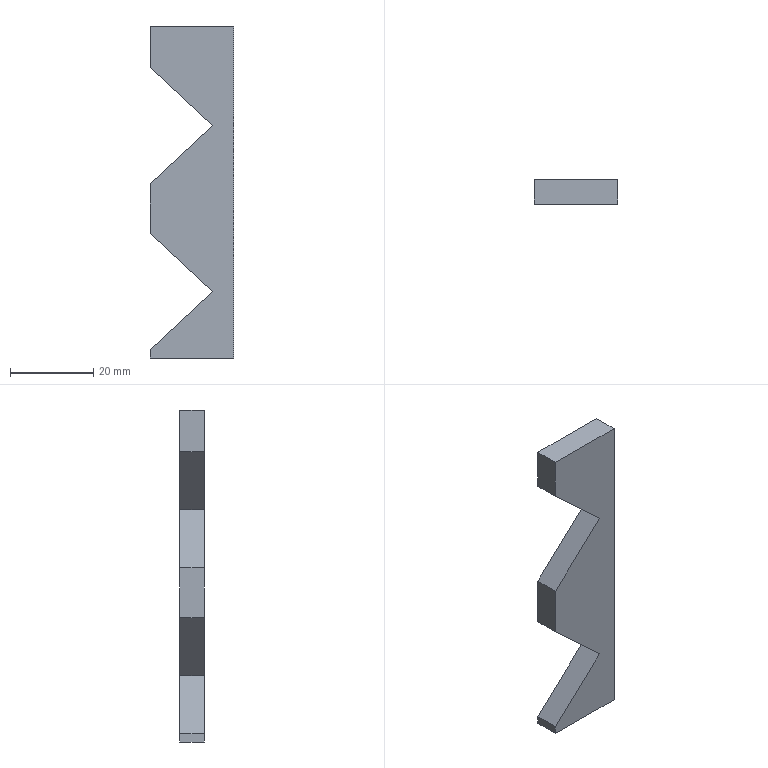Component | NX | V_SLIDER | 1 solid | 12 faces | box 20 x 6 x 80 mm | volume 7082 mm3 | plane 12
STEP:
#1=CARTESIAN_POINT('',(0.,0.,0.));
#2=DIRECTION('',(0.,0.,1.));
#3=DIRECTION('',(1.,0.,0.));
#4=AXIS2_PLACEMENT_3D('',#1,#2,#3);
#5=CARTESIAN_POINT('',(65.,-18.,99.));
#6=VERTEX_POINT('',#5);
#7=CARTESIAN_POINT('',(65.,-18.,19.));
#8=VERTEX_POINT('',#7);
#9=CARTESIAN_POINT('',(65.,-18.,99.));
#10=DIRECTION('',(0.,0.,-1.));
#11=VECTOR('',#10,1.);
#12=LINE('',#9,#11);
#13=CARTESIAN_POINT('',(65.,-12.,99.));
#14=DIRECTION('',(-1.,0.,0.));
#15=DIRECTION('',(0.,-1.,0.));
#16=AXIS2_PLACEMENT_3D('',#13,#14,#15);
#17=PLANE('',#16);
#18=CARTESIAN_POINT('',(6.,0.));
#19=DIRECTION('',(0.,-1.));
#20=VECTOR('',#19,1.);
#21=LINE('',#18,#20);
#22=(GEOMETRIC_REPRESENTATION_CONTEXT(2)PARAMETRIC_REPRESENTATION_CONTEXT()REPRESENTATION_CONTEXT('',''));
#23=DEFINITIONAL_REPRESENTATION('',(#21),#22);
#24=PCURVE('',#17,#23);
#25=CARTESIAN_POINT('',(65.,-18.,19.));
#26=DIRECTION('',(0.,1.,0.));
#27=DIRECTION('',(-1.,0.,0.));
#28=AXIS2_PLACEMENT_3D('',#25,#26,#27);
#29=PLANE('',#28);
#30=CARTESIAN_POINT('',(0.,80.));
#31=DIRECTION('',(0.,-1.));
#32=VECTOR('',#31,1.);
#33=LINE('',#30,#32);
#34=(GEOMETRIC_REPRESENTATION_CONTEXT(2)PARAMETRIC_REPRESENTATION_CONTEXT()REPRESENTATION_CONTEXT('',''));
#35=DEFINITIONAL_REPRESENTATION('',(#33),#34);
#36=PCURVE('',#29,#35);
#37=SURFACE_CURVE('',#12,(#24,#36),.PCURVE_S1.);
#38=EDGE_CURVE('',#6,#8,#37,.T.);
#39=ORIENTED_EDGE('',*,*,#38,.T.);
#40=CARTESIAN_POINT('',(65.,-12.,19.));
#41=VERTEX_POINT('',#40);
#42=CARTESIAN_POINT('',(65.,-12.,19.));
#43=DIRECTION('',(0.,-1.,0.));
#44=VECTOR('',#43,1.);
#45=LINE('',#42,#44);
#46=CARTESIAN_POINT('',(0.,-80.));
#47=DIRECTION('',(1.,0.));
#48=VECTOR('',#47,1.);
#49=LINE('',#46,#48);
#50=(GEOMETRIC_REPRESENTATION_CONTEXT(2)PARAMETRIC_REPRESENTATION_CONTEXT()REPRESENTATION_CONTEXT('',''));
#51=DEFINITIONAL_REPRESENTATION('',(#49),#50);
#52=PCURVE('',#17,#51);
#53=CARTESIAN_POINT('',(65.,-12.,19.));
#54=DIRECTION('',(-0.,0.,1.));
#55=DIRECTION('',(1.,0.,0.));
#56=AXIS2_PLACEMENT_3D('',#53,#54,#55);
#57=PLANE('',#56);
#58=CARTESIAN_POINT('',(0.,0.));
#59=DIRECTION('',(0.,-1.));
#60=VECTOR('',#59,1.);
#61=LINE('',#58,#60);
#62=(GEOMETRIC_REPRESENTATION_CONTEXT(2)PARAMETRIC_REPRESENTATION_CONTEXT()REPRESENTATION_CONTEXT('',''));
#63=DEFINITIONAL_REPRESENTATION('',(#61),#62);
#64=PCURVE('',#57,#63);
#65=SURFACE_CURVE('',#45,(#52,#64),.PCURVE_S1.);
#66=EDGE_CURVE('',#41,#8,#65,.T.);
#67=ORIENTED_EDGE('',*,*,#66,.F.);
#68=CARTESIAN_POINT('',(65.,-12.,99.));
#69=VERTEX_POINT('',#68);
#70=CARTESIAN_POINT('',(65.,-12.,99.));
#71=DIRECTION('',(0.,0.,-1.));
#72=VECTOR('',#71,1.);
#73=LINE('',#70,#72);
#74=CARTESIAN_POINT('',(0.,0.));
#75=DIRECTION('',(0.,-1.));
#76=VECTOR('',#75,1.);
#77=LINE('',#74,#76);
#78=(GEOMETRIC_REPRESENTATION_CONTEXT(2)PARAMETRIC_REPRESENTATION_CONTEXT()REPRESENTATION_CONTEXT('',''));
#79=DEFINITIONAL_REPRESENTATION('',(#77),#78);
#80=PCURVE('',#17,#79);
#81=CARTESIAN_POINT('',(65.,-12.,19.));
#82=DIRECTION('',(0.,1.,0.));
#83=DIRECTION('',(-1.,0.,0.));
#84=AXIS2_PLACEMENT_3D('',#81,#82,#83);
#85=PLANE('',#84);
#86=CARTESIAN_POINT('',(0.,80.));
#87=DIRECTION('',(0.,-1.));
#88=VECTOR('',#87,1.);
#89=LINE('',#86,#88);
#90=(GEOMETRIC_REPRESENTATION_CONTEXT(2)PARAMETRIC_REPRESENTATION_CONTEXT()REPRESENTATION_CONTEXT('',''));
#91=DEFINITIONAL_REPRESENTATION('',(#89),#90);
#92=PCURVE('',#85,#91);
#93=SURFACE_CURVE('',#73,(#80,#92),.PCURVE_S1.);
#94=EDGE_CURVE('',#69,#41,#93,.T.);
#95=ORIENTED_EDGE('',*,*,#94,.F.);
#96=CARTESIAN_POINT('',(65.,-12.,99.));
#97=DIRECTION('',(0.,-1.,0.));
#98=VECTOR('',#97,1.);
#99=LINE('',#96,#98);
#100=CARTESIAN_POINT('',(0.,0.));
#101=DIRECTION('',(1.,0.));
#102=VECTOR('',#101,1.);
#103=LINE('',#100,#102);
#104=(GEOMETRIC_REPRESENTATION_CONTEXT(2)PARAMETRIC_REPRESENTATION_CONTEXT()REPRESENTATION_CONTEXT('',''));
#105=DEFINITIONAL_REPRESENTATION('',(#103),#104);
#106=PCURVE('',#17,#105);
#107=CARTESIAN_POINT('',(45.,-12.,99.));
#108=DIRECTION('',(0.,0.,-1.));
#109=DIRECTION('',(0.,-1.,0.));
#110=AXIS2_PLACEMENT_3D('',#107,#108,#109);
#111=PLANE('',#110);
#112=CARTESIAN_POINT('',(0.,-20.));
#113=DIRECTION('',(1.,0.));
#114=VECTOR('',#113,1.);
#115=LINE('',#112,#114);
#116=(GEOMETRIC_REPRESENTATION_CONTEXT(2)PARAMETRIC_REPRESENTATION_CONTEXT()REPRESENTATION_CONTEXT('',''));
#117=DEFINITIONAL_REPRESENTATION('',(#115),#116);
#118=PCURVE('',#111,#117);
#119=SURFACE_CURVE('',#99,(#106,#118),.PCURVE_S1.);
#120=EDGE_CURVE('',#69,#6,#119,.T.);
#121=ORIENTED_EDGE('',*,*,#120,.T.);
#122=EDGE_LOOP('',(#39,#67,#95,#121));
#123=FACE_BOUND('',#122,.T.);
#124=ADVANCED_FACE('',(#123),#17,.F.);
#125=CARTESIAN_POINT('',(45.,-18.,19.));
#126=VERTEX_POINT('',#125);
#127=CARTESIAN_POINT('',(65.,-18.,19.));
#128=DIRECTION('',(-1.,0.,-0.));
#129=VECTOR('',#128,1.);
#130=LINE('',#127,#129);
#131=CARTESIAN_POINT('',(0.,-6.));
#132=DIRECTION('',(-1.,0.));
#133=VECTOR('',#132,1.);
#134=LINE('',#131,#133);
#135=(GEOMETRIC_REPRESENTATION_CONTEXT(2)PARAMETRIC_REPRESENTATION_CONTEXT()REPRESENTATION_CONTEXT('',''));
#136=DEFINITIONAL_REPRESENTATION('',(#134),#135);
#137=PCURVE('',#57,#136);
#138=CARTESIAN_POINT('',(0.,0.));
#139=DIRECTION('',(1.,-0.));
#140=VECTOR('',#139,1.);
#141=LINE('',#138,#140);
#142=(GEOMETRIC_REPRESENTATION_CONTEXT(2)PARAMETRIC_REPRESENTATION_CONTEXT()REPRESENTATION_CONTEXT('',''));
#143=DEFINITIONAL_REPRESENTATION('',(#141),#142);
#144=PCURVE('',#29,#143);
#145=SURFACE_CURVE('',#130,(#137,#144),.PCURVE_S1.);
#146=EDGE_CURVE('',#8,#126,#145,.T.);
#147=ORIENTED_EDGE('',*,*,#146,.T.);
#148=CARTESIAN_POINT('',(45.,-12.,19.));
#149=VERTEX_POINT('',#148);
#150=CARTESIAN_POINT('',(45.,-12.,19.));
#151=DIRECTION('',(0.,-1.,0.));
#152=VECTOR('',#151,1.);
#153=LINE('',#150,#152);
#154=CARTESIAN_POINT('',(-20.,0.));
#155=DIRECTION('',(0.,-1.));
#156=VECTOR('',#155,1.);
#157=LINE('',#154,#156);
#158=(GEOMETRIC_REPRESENTATION_CONTEXT(2)PARAMETRIC_REPRESENTATION_CONTEXT()REPRESENTATION_CONTEXT('',''));
#159=DEFINITIONAL_REPRESENTATION('',(#157),#158);
#160=PCURVE('',#57,#159);
#161=CARTESIAN_POINT('',(45.,-12.,19.));
#162=DIRECTION('',(1.,0.,0.));
#163=DIRECTION('',(0.,1.,0.));
#164=AXIS2_PLACEMENT_3D('',#161,#162,#163);
#165=PLANE('',#164);
#166=CARTESIAN_POINT('',(0.,0.));
#167=DIRECTION('',(-1.,0.));
#168=VECTOR('',#167,1.);
#169=LINE('',#166,#168);
#170=(GEOMETRIC_REPRESENTATION_CONTEXT(2)PARAMETRIC_REPRESENTATION_CONTEXT()REPRESENTATION_CONTEXT('',''));
#171=DEFINITIONAL_REPRESENTATION('',(#169),#170);
#172=PCURVE('',#165,#171);
#173=SURFACE_CURVE('',#153,(#160,#172),.PCURVE_S1.);
#174=EDGE_CURVE('',#149,#126,#173,.T.);
#175=ORIENTED_EDGE('',*,*,#174,.F.);
#176=CARTESIAN_POINT('',(65.,-12.,19.));
#177=DIRECTION('',(-1.,0.,-0.));
#178=VECTOR('',#177,1.);
#179=LINE('',#176,#178);
#180=CARTESIAN_POINT('',(0.,0.));
#181=DIRECTION('',(-1.,0.));
#182=VECTOR('',#181,1.);
#183=LINE('',#180,#182);
#184=(GEOMETRIC_REPRESENTATION_CONTEXT(2)PARAMETRIC_REPRESENTATION_CONTEXT()REPRESENTATION_CONTEXT('',''));
#185=DEFINITIONAL_REPRESENTATION('',(#183),#184);
#186=PCURVE('',#57,#185);
#187=CARTESIAN_POINT('',(0.,0.));
#188=DIRECTION('',(1.,-0.));
#189=VECTOR('',#188,1.);
#190=LINE('',#187,#189);
#191=(GEOMETRIC_REPRESENTATION_CONTEXT(2)PARAMETRIC_REPRESENTATION_CONTEXT()REPRESENTATION_CONTEXT('',''));
#192=DEFINITIONAL_REPRESENTATION('',(#190),#191);
#193=PCURVE('',#85,#192);
#194=SURFACE_CURVE('',#179,(#186,#193),.PCURVE_S1.);
#195=EDGE_CURVE('',#41,#149,#194,.T.);
#196=ORIENTED_EDGE('',*,*,#195,.F.);
#197=ORIENTED_EDGE('',*,*,#66,.T.);
#198=EDGE_LOOP('',(#147,#175,#196,#197));
#199=FACE_BOUND('',#198,.T.);
#200=ADVANCED_FACE('',(#199),#57,.F.);
#201=CARTESIAN_POINT('',(45.,-18.,21.012));
#202=VERTEX_POINT('',#201);
#203=CARTESIAN_POINT('',(45.,-18.,19.));
#204=DIRECTION('',(0.,0.,1.));
#205=VECTOR('',#204,1.);
#206=LINE('',#203,#205);
#207=CARTESIAN_POINT('',(-6.,0.));
#208=DIRECTION('',(0.,1.));
#209=VECTOR('',#208,1.);
#210=LINE('',#207,#209);
#211=(GEOMETRIC_REPRESENTATION_CONTEXT(2)PARAMETRIC_REPRESENTATION_CONTEXT()REPRESENTATION_CONTEXT('',''));
#212=DEFINITIONAL_REPRESENTATION('',(#210),#211);
#213=PCURVE('',#165,#212);
#214=CARTESIAN_POINT('',(20.,0.));
#215=DIRECTION('',(0.,1.));
#216=VECTOR('',#215,1.);
#217=LINE('',#214,#216);
#218=(GEOMETRIC_REPRESENTATION_CONTEXT(2)PARAMETRIC_REPRESENTATION_CONTEXT()REPRESENTATION_CONTEXT('',''));
#219=DEFINITIONAL_REPRESENTATION('',(#217),#218);
#220=PCURVE('',#29,#219);
#221=SURFACE_CURVE('',#206,(#213,#220),.PCURVE_S1.);
#222=EDGE_CURVE('',#126,#202,#221,.T.);
#223=ORIENTED_EDGE('',*,*,#222,.T.);
#224=CARTESIAN_POINT('',(45.,-12.,21.012));
#225=VERTEX_POINT('',#224);
#226=CARTESIAN_POINT('',(45.,-12.,21.012));
#227=DIRECTION('',(0.,-1.,0.));
#228=VECTOR('',#227,1.);
#229=LINE('',#226,#228);
#230=CARTESIAN_POINT('',(0.,2.012));
#231=DIRECTION('',(-1.,0.));
#232=VECTOR('',#231,1.);
#233=LINE('',#230,#232);
#234=(GEOMETRIC_REPRESENTATION_CONTEXT(2)PARAMETRIC_REPRESENTATION_CONTEXT()REPRESENTATION_CONTEXT('',''));
#235=DEFINITIONAL_REPRESENTATION('',(#233),#234);
#236=PCURVE('',#165,#235);
#237=CARTESIAN_POINT('',(45.,-12.,21.012));
#238=DIRECTION('',(0.682,0.,-0.7314));
#239=DIRECTION('',(-0.7314,0.,-0.682));
#240=AXIS2_PLACEMENT_3D('',#237,#238,#239);
#241=PLANE('',#240);
#242=CARTESIAN_POINT('',(0.,0.));
#243=DIRECTION('',(0.,-1.));
#244=VECTOR('',#243,1.);
#245=LINE('',#242,#244);
#246=(GEOMETRIC_REPRESENTATION_CONTEXT(2)PARAMETRIC_REPRESENTATION_CONTEXT()REPRESENTATION_CONTEXT('',''));
#247=DEFINITIONAL_REPRESENTATION('',(#245),#246);
#248=PCURVE('',#241,#247);
#249=SURFACE_CURVE('',#229,(#236,#248),.PCURVE_S1.);
#250=EDGE_CURVE('',#225,#202,#249,.T.);
#251=ORIENTED_EDGE('',*,*,#250,.F.);
#252=CARTESIAN_POINT('',(45.,-12.,19.));
#253=DIRECTION('',(0.,0.,1.));
#254=VECTOR('',#253,1.);
#255=LINE('',#252,#254);
#256=CARTESIAN_POINT('',(0.,0.));
#257=DIRECTION('',(0.,1.));
#258=VECTOR('',#257,1.);
#259=LINE('',#256,#258);
#260=(GEOMETRIC_REPRESENTATION_CONTEXT(2)PARAMETRIC_REPRESENTATION_CONTEXT()REPRESENTATION_CONTEXT('',''));
#261=DEFINITIONAL_REPRESENTATION('',(#259),#260);
#262=PCURVE('',#165,#261);
#263=CARTESIAN_POINT('',(20.,0.));
#264=DIRECTION('',(0.,1.));
#265=VECTOR('',#264,1.);
#266=LINE('',#263,#265);
#267=(GEOMETRIC_REPRESENTATION_CONTEXT(2)PARAMETRIC_REPRESENTATION_CONTEXT()REPRESENTATION_CONTEXT('',''));
#268=DEFINITIONAL_REPRESENTATION('',(#266),#267);
#269=PCURVE('',#85,#268);
#270=SURFACE_CURVE('',#255,(#262,#269),.PCURVE_S1.);
#271=EDGE_CURVE('',#149,#225,#270,.T.);
#272=ORIENTED_EDGE('',*,*,#271,.F.);
#273=ORIENTED_EDGE('',*,*,#174,.T.);
#274=EDGE_LOOP('',(#223,#251,#272,#273));
#275=FACE_BOUND('',#274,.T.);
#276=ADVANCED_FACE('',(#275),#165,.F.);
#277=CARTESIAN_POINT('',(60.,-18.,35.));
#278=VERTEX_POINT('',#277);
#279=CARTESIAN_POINT('',(45.,-18.,21.012));
#280=DIRECTION('',(0.7314,0.,0.682));
#281=VECTOR('',#280,1.);
#282=LINE('',#279,#281);
#283=CARTESIAN_POINT('',(0.,-6.));
#284=DIRECTION('',(-1.,0.));
#285=VECTOR('',#284,1.);
#286=LINE('',#283,#285);
#287=(GEOMETRIC_REPRESENTATION_CONTEXT(2)PARAMETRIC_REPRESENTATION_CONTEXT()REPRESENTATION_CONTEXT('',''));
#288=DEFINITIONAL_REPRESENTATION('',(#286),#287);
#289=PCURVE('',#241,#288);
#290=CARTESIAN_POINT('',(20.,2.012));
#291=DIRECTION('',(-0.7314,0.682));
#292=VECTOR('',#291,1.);
#293=LINE('',#290,#292);
#294=(GEOMETRIC_REPRESENTATION_CONTEXT(2)PARAMETRIC_REPRESENTATION_CONTEXT()REPRESENTATION_CONTEXT('',''));
#295=DEFINITIONAL_REPRESENTATION('',(#293),#294);
#296=PCURVE('',#29,#295);
#297=SURFACE_CURVE('',#282,(#289,#296),.PCURVE_S1.);
#298=EDGE_CURVE('',#202,#278,#297,.T.);
#299=ORIENTED_EDGE('',*,*,#298,.T.);
#300=CARTESIAN_POINT('',(60.,-12.,35.));
#301=VERTEX_POINT('',#300);
#302=CARTESIAN_POINT('',(60.,-12.,35.));
#303=DIRECTION('',(0.,-1.,0.));
#304=VECTOR('',#303,1.);
#305=LINE('',#302,#304);
#306=CARTESIAN_POINT('',(-20.51,0.));
#307=DIRECTION('',(0.,-1.));
#308=VECTOR('',#307,1.);
#309=LINE('',#306,#308);
#310=(GEOMETRIC_REPRESENTATION_CONTEXT(2)PARAMETRIC_REPRESENTATION_CONTEXT()REPRESENTATION_CONTEXT('',''));
#311=DEFINITIONAL_REPRESENTATION('',(#309),#310);
#312=PCURVE('',#241,#311);
#313=CARTESIAN_POINT('',(60.,-12.,35.));
#314=DIRECTION('',(0.682,0.,0.7314));
#315=DIRECTION('',(0.7314,0.,-0.682));
#316=AXIS2_PLACEMENT_3D('',#313,#314,#315);
#317=PLANE('',#316);
#318=CARTESIAN_POINT('',(0.,0.));
#319=DIRECTION('',(0.,-1.));
#320=VECTOR('',#319,1.);
#321=LINE('',#318,#320);
#322=(GEOMETRIC_REPRESENTATION_CONTEXT(2)PARAMETRIC_REPRESENTATION_CONTEXT()REPRESENTATION_CONTEXT('',''));
#323=DEFINITIONAL_REPRESENTATION('',(#321),#322);
#324=PCURVE('',#317,#323);
#325=SURFACE_CURVE('',#305,(#312,#324),.PCURVE_S1.);
#326=EDGE_CURVE('',#301,#278,#325,.T.);
#327=ORIENTED_EDGE('',*,*,#326,.F.);
#328=CARTESIAN_POINT('',(45.,-12.,21.012));
#329=DIRECTION('',(0.7314,0.,0.682));
#330=VECTOR('',#329,1.);
#331=LINE('',#328,#330);
#332=CARTESIAN_POINT('',(0.,0.));
#333=DIRECTION('',(-1.,0.));
#334=VECTOR('',#333,1.);
#335=LINE('',#332,#334);
#336=(GEOMETRIC_REPRESENTATION_CONTEXT(2)PARAMETRIC_REPRESENTATION_CONTEXT()REPRESENTATION_CONTEXT('',''));
#337=DEFINITIONAL_REPRESENTATION('',(#335),#336);
#338=PCURVE('',#241,#337);
#339=CARTESIAN_POINT('',(20.,2.012));
#340=DIRECTION('',(-0.7314,0.682));
#341=VECTOR('',#340,1.);
#342=LINE('',#339,#341);
#343=(GEOMETRIC_REPRESENTATION_CONTEXT(2)PARAMETRIC_REPRESENTATION_CONTEXT()REPRESENTATION_CONTEXT('',''));
#344=DEFINITIONAL_REPRESENTATION('',(#342),#343);
#345=PCURVE('',#85,#344);
#346=SURFACE_CURVE('',#331,(#338,#345),.PCURVE_S1.);
#347=EDGE_CURVE('',#225,#301,#346,.T.);
#348=ORIENTED_EDGE('',*,*,#347,.F.);
#349=ORIENTED_EDGE('',*,*,#250,.T.);
#350=EDGE_LOOP('',(#299,#327,#348,#349));
#351=FACE_BOUND('',#350,.T.);
#352=ADVANCED_FACE('',(#351),#241,.F.);
#353=CARTESIAN_POINT('',(45.,-18.,48.988));
#354=VERTEX_POINT('',#353);
#355=CARTESIAN_POINT('',(60.,-18.,35.));
#356=DIRECTION('',(-0.7314,0.,0.682));
#357=VECTOR('',#356,1.);
#358=LINE('',#355,#357);
#359=CARTESIAN_POINT('',(0.,-6.));
#360=DIRECTION('',(-1.,0.));
#361=VECTOR('',#360,1.);
#362=LINE('',#359,#361);
#363=(GEOMETRIC_REPRESENTATION_CONTEXT(2)PARAMETRIC_REPRESENTATION_CONTEXT()REPRESENTATION_CONTEXT('',''));
#364=DEFINITIONAL_REPRESENTATION('',(#362),#363);
#365=PCURVE('',#317,#364);
#366=CARTESIAN_POINT('',(5.,16.));
#367=DIRECTION('',(0.7314,0.682));
#368=VECTOR('',#367,1.);
#369=LINE('',#366,#368);
#370=(GEOMETRIC_REPRESENTATION_CONTEXT(2)PARAMETRIC_REPRESENTATION_CONTEXT()REPRESENTATION_CONTEXT('',''));
#371=DEFINITIONAL_REPRESENTATION('',(#369),#370);
#372=PCURVE('',#29,#371);
#373=SURFACE_CURVE('',#358,(#365,#372),.PCURVE_S1.);
#374=EDGE_CURVE('',#278,#354,#373,.T.);
#375=ORIENTED_EDGE('',*,*,#374,.T.);
#376=CARTESIAN_POINT('',(45.,-12.,48.988));
#377=VERTEX_POINT('',#376);
#378=CARTESIAN_POINT('',(45.,-12.,48.988));
#379=DIRECTION('',(0.,-1.,0.));
#380=VECTOR('',#379,1.);
#381=LINE('',#378,#380);
#382=CARTESIAN_POINT('',(-20.51,0.));
#383=DIRECTION('',(0.,-1.));
#384=VECTOR('',#383,1.);
#385=LINE('',#382,#384);
#386=(GEOMETRIC_REPRESENTATION_CONTEXT(2)PARAMETRIC_REPRESENTATION_CONTEXT()REPRESENTATION_CONTEXT('',''));
#387=DEFINITIONAL_REPRESENTATION('',(#385),#386);
#388=PCURVE('',#317,#387);
#389=CARTESIAN_POINT('',(45.,-12.,48.988));
#390=DIRECTION('',(1.,0.,-0.));
#391=DIRECTION('',(-0.,0.,-1.));
#392=AXIS2_PLACEMENT_3D('',#389,#390,#391);
#393=PLANE('',#392);
#394=CARTESIAN_POINT('',(0.,0.));
#395=DIRECTION('',(0.,-1.));
#396=VECTOR('',#395,1.);
#397=LINE('',#394,#396);
#398=(GEOMETRIC_REPRESENTATION_CONTEXT(2)PARAMETRIC_REPRESENTATION_CONTEXT()REPRESENTATION_CONTEXT('',''));
#399=DEFINITIONAL_REPRESENTATION('',(#397),#398);
#400=PCURVE('',#393,#399);
#401=SURFACE_CURVE('',#381,(#388,#400),.PCURVE_S1.);
#402=EDGE_CURVE('',#377,#354,#401,.T.);
#403=ORIENTED_EDGE('',*,*,#402,.F.);
#404=CARTESIAN_POINT('',(60.,-12.,35.));
#405=DIRECTION('',(-0.7314,0.,0.682));
#406=VECTOR('',#405,1.);
#407=LINE('',#404,#406);
#408=CARTESIAN_POINT('',(0.,0.));
#409=DIRECTION('',(-1.,0.));
#410=VECTOR('',#409,1.);
#411=LINE('',#408,#410);
#412=(GEOMETRIC_REPRESENTATION_CONTEXT(2)PARAMETRIC_REPRESENTATION_CONTEXT()REPRESENTATION_CONTEXT('',''));
#413=DEFINITIONAL_REPRESENTATION('',(#411),#412);
#414=PCURVE('',#317,#413);
#415=CARTESIAN_POINT('',(5.,16.));
#416=DIRECTION('',(0.7314,0.682));
#417=VECTOR('',#416,1.);
#418=LINE('',#415,#417);
#419=(GEOMETRIC_REPRESENTATION_CONTEXT(2)PARAMETRIC_REPRESENTATION_CONTEXT()REPRESENTATION_CONTEXT('',''));
#420=DEFINITIONAL_REPRESENTATION('',(#418),#419);
#421=PCURVE('',#85,#420);
#422=SURFACE_CURVE('',#407,(#414,#421),.PCURVE_S1.);
#423=EDGE_CURVE('',#301,#377,#422,.T.);
#424=ORIENTED_EDGE('',*,*,#423,.F.);
#425=ORIENTED_EDGE('',*,*,#326,.T.);
#426=EDGE_LOOP('',(#375,#403,#424,#425));
#427=FACE_BOUND('',#426,.T.);
#428=ADVANCED_FACE('',(#427),#317,.F.);
#429=CARTESIAN_POINT('',(45.,-18.,61.012));
#430=VERTEX_POINT('',#429);
#431=CARTESIAN_POINT('',(45.,-18.,48.988));
#432=DIRECTION('',(0.,0.,1.));
#433=VECTOR('',#432,1.);
#434=LINE('',#431,#433);
#435=CARTESIAN_POINT('',(0.,-6.));
#436=DIRECTION('',(-1.,0.));
#437=VECTOR('',#436,1.);
#438=LINE('',#435,#437);
#439=(GEOMETRIC_REPRESENTATION_CONTEXT(2)PARAMETRIC_REPRESENTATION_CONTEXT()REPRESENTATION_CONTEXT('',''));
#440=DEFINITIONAL_REPRESENTATION('',(#438),#439);
#441=PCURVE('',#393,#440);
#442=CARTESIAN_POINT('',(20.,29.988));
#443=DIRECTION('',(-0.,1.));
#444=VECTOR('',#443,1.);
#445=LINE('',#442,#444);
#446=(GEOMETRIC_REPRESENTATION_CONTEXT(2)PARAMETRIC_REPRESENTATION_CONTEXT()REPRESENTATION_CONTEXT('',''));
#447=DEFINITIONAL_REPRESENTATION('',(#445),#446);
#448=PCURVE('',#29,#447);
#449=SURFACE_CURVE('',#434,(#441,#448),.PCURVE_S1.);
#450=EDGE_CURVE('',#354,#430,#449,.T.);
#451=ORIENTED_EDGE('',*,*,#450,.T.);
#452=CARTESIAN_POINT('',(45.,-12.,61.012));
#453=VERTEX_POINT('',#452);
#454=CARTESIAN_POINT('',(45.,-12.,61.012));
#455=DIRECTION('',(0.,-1.,0.));
#456=VECTOR('',#455,1.);
#457=LINE('',#454,#456);
#458=CARTESIAN_POINT('',(-12.025,0.));
#459=DIRECTION('',(0.,-1.));
#460=VECTOR('',#459,1.);
#461=LINE('',#458,#460);
#462=(GEOMETRIC_REPRESENTATION_CONTEXT(2)PARAMETRIC_REPRESENTATION_CONTEXT()REPRESENTATION_CONTEXT('',''));
#463=DEFINITIONAL_REPRESENTATION('',(#461),#462);
#464=PCURVE('',#393,#463);
#465=CARTESIAN_POINT('',(45.,-12.,61.012));
#466=DIRECTION('',(0.682,0.,-0.7314));
#467=DIRECTION('',(-0.7314,0.,-0.682));
#468=AXIS2_PLACEMENT_3D('',#465,#466,#467);
#469=PLANE('',#468);
#470=CARTESIAN_POINT('',(0.,0.));
#471=DIRECTION('',(0.,-1.));
#472=VECTOR('',#471,1.);
#473=LINE('',#470,#472);
#474=(GEOMETRIC_REPRESENTATION_CONTEXT(2)PARAMETRIC_REPRESENTATION_CONTEXT()REPRESENTATION_CONTEXT('',''));
#475=DEFINITIONAL_REPRESENTATION('',(#473),#474);
#476=PCURVE('',#469,#475);
#477=SURFACE_CURVE('',#457,(#464,#476),.PCURVE_S1.);
#478=EDGE_CURVE('',#453,#430,#477,.T.);
#479=ORIENTED_EDGE('',*,*,#478,.F.);
#480=CARTESIAN_POINT('',(45.,-12.,48.988));
#481=DIRECTION('',(0.,0.,1.));
#482=VECTOR('',#481,1.);
#483=LINE('',#480,#482);
#484=CARTESIAN_POINT('',(0.,0.));
#485=DIRECTION('',(-1.,0.));
#486=VECTOR('',#485,1.);
#487=LINE('',#484,#486);
#488=(GEOMETRIC_REPRESENTATION_CONTEXT(2)PARAMETRIC_REPRESENTATION_CONTEXT()REPRESENTATION_CONTEXT('',''));
#489=DEFINITIONAL_REPRESENTATION('',(#487),#488);
#490=PCURVE('',#393,#489);
#491=CARTESIAN_POINT('',(20.,29.988));
#492=DIRECTION('',(-0.,1.));
#493=VECTOR('',#492,1.);
#494=LINE('',#491,#493);
#495=(GEOMETRIC_REPRESENTATION_CONTEXT(2)PARAMETRIC_REPRESENTATION_CONTEXT()REPRESENTATION_CONTEXT('',''));
#496=DEFINITIONAL_REPRESENTATION('',(#494),#495);
#497=PCURVE('',#85,#496);
#498=SURFACE_CURVE('',#483,(#490,#497),.PCURVE_S1.);
#499=EDGE_CURVE('',#377,#453,#498,.T.);
#500=ORIENTED_EDGE('',*,*,#499,.F.);
#501=ORIENTED_EDGE('',*,*,#402,.T.);
#502=EDGE_LOOP('',(#451,#479,#500,#501));
#503=FACE_BOUND('',#502,.T.);
#504=ADVANCED_FACE('',(#503),#393,.F.);
#505=CARTESIAN_POINT('',(60.,-18.,75.));
#506=VERTEX_POINT('',#505);
#507=CARTESIAN_POINT('',(45.,-18.,61.012));
#508=DIRECTION('',(0.7314,0.,0.682));
#509=VECTOR('',#508,1.);
#510=LINE('',#507,#509);
#511=CARTESIAN_POINT('',(0.,-6.));
#512=DIRECTION('',(-1.,0.));
#513=VECTOR('',#512,1.);
#514=LINE('',#511,#513);
#515=(GEOMETRIC_REPRESENTATION_CONTEXT(2)PARAMETRIC_REPRESENTATION_CONTEXT()REPRESENTATION_CONTEXT('',''));
#516=DEFINITIONAL_REPRESENTATION('',(#514),#515);
#517=PCURVE('',#469,#516);
#518=CARTESIAN_POINT('',(20.,42.012));
#519=DIRECTION('',(-0.7314,0.682));
#520=VECTOR('',#519,1.);
#521=LINE('',#518,#520);
#522=(GEOMETRIC_REPRESENTATION_CONTEXT(2)PARAMETRIC_REPRESENTATION_CONTEXT()REPRESENTATION_CONTEXT('',''));
#523=DEFINITIONAL_REPRESENTATION('',(#521),#522);
#524=PCURVE('',#29,#523);
#525=SURFACE_CURVE('',#510,(#517,#524),.PCURVE_S1.);
#526=EDGE_CURVE('',#430,#506,#525,.T.);
#527=ORIENTED_EDGE('',*,*,#526,.T.);
#528=CARTESIAN_POINT('',(60.,-12.,75.));
#529=VERTEX_POINT('',#528);
#530=CARTESIAN_POINT('',(60.,-12.,75.));
#531=DIRECTION('',(0.,-1.,0.));
#532=VECTOR('',#531,1.);
#533=LINE('',#530,#532);
#534=CARTESIAN_POINT('',(-20.51,0.));
#535=DIRECTION('',(0.,-1.));
#536=VECTOR('',#535,1.);
#537=LINE('',#534,#536);
#538=(GEOMETRIC_REPRESENTATION_CONTEXT(2)PARAMETRIC_REPRESENTATION_CONTEXT()REPRESENTATION_CONTEXT('',''));
#539=DEFINITIONAL_REPRESENTATION('',(#537),#538);
#540=PCURVE('',#469,#539);
#541=CARTESIAN_POINT('',(60.,-12.,75.));
#542=DIRECTION('',(0.682,0.,0.7314));
#543=DIRECTION('',(0.7314,0.,-0.682));
#544=AXIS2_PLACEMENT_3D('',#541,#542,#543);
#545=PLANE('',#544);
#546=CARTESIAN_POINT('',(0.,0.));
#547=DIRECTION('',(0.,-1.));
#548=VECTOR('',#547,1.);
#549=LINE('',#546,#548);
#550=(GEOMETRIC_REPRESENTATION_CONTEXT(2)PARAMETRIC_REPRESENTATION_CONTEXT()REPRESENTATION_CONTEXT('',''));
#551=DEFINITIONAL_REPRESENTATION('',(#549),#550);
#552=PCURVE('',#545,#551);
#553=SURFACE_CURVE('',#533,(#540,#552),.PCURVE_S1.);
#554=EDGE_CURVE('',#529,#506,#553,.T.);
#555=ORIENTED_EDGE('',*,*,#554,.F.);
#556=CARTESIAN_POINT('',(45.,-12.,61.012));
#557=DIRECTION('',(0.7314,0.,0.682));
#558=VECTOR('',#557,1.);
#559=LINE('',#556,#558);
#560=CARTESIAN_POINT('',(0.,0.));
#561=DIRECTION('',(-1.,0.));
#562=VECTOR('',#561,1.);
#563=LINE('',#560,#562);
#564=(GEOMETRIC_REPRESENTATION_CONTEXT(2)PARAMETRIC_REPRESENTATION_CONTEXT()REPRESENTATION_CONTEXT('',''));
#565=DEFINITIONAL_REPRESENTATION('',(#563),#564);
#566=PCURVE('',#469,#565);
#567=CARTESIAN_POINT('',(20.,42.012));
#568=DIRECTION('',(-0.7314,0.682));
#569=VECTOR('',#568,1.);
#570=LINE('',#567,#569);
#571=(GEOMETRIC_REPRESENTATION_CONTEXT(2)PARAMETRIC_REPRESENTATION_CONTEXT()REPRESENTATION_CONTEXT('',''));
#572=DEFINITIONAL_REPRESENTATION('',(#570),#571);
#573=PCURVE('',#85,#572);
#574=SURFACE_CURVE('',#559,(#566,#573),.PCURVE_S1.);
#575=EDGE_CURVE('',#453,#529,#574,.T.);
#576=ORIENTED_EDGE('',*,*,#575,.F.);
#577=ORIENTED_EDGE('',*,*,#478,.T.);
#578=EDGE_LOOP('',(#527,#555,#576,#577));
#579=FACE_BOUND('',#578,.T.);
#580=ADVANCED_FACE('',(#579),#469,.F.);
#581=CARTESIAN_POINT('',(45.,-18.,88.988));
#582=VERTEX_POINT('',#581);
#583=CARTESIAN_POINT('',(60.,-18.,75.));
#584=DIRECTION('',(-0.7314,0.,0.682));
#585=VECTOR('',#584,1.);
#586=LINE('',#583,#585);
#587=CARTESIAN_POINT('',(0.,-6.));
#588=DIRECTION('',(-1.,0.));
#589=VECTOR('',#588,1.);
#590=LINE('',#587,#589);
#591=(GEOMETRIC_REPRESENTATION_CONTEXT(2)PARAMETRIC_REPRESENTATION_CONTEXT()REPRESENTATION_CONTEXT('',''));
#592=DEFINITIONAL_REPRESENTATION('',(#590),#591);
#593=PCURVE('',#545,#592);
#594=CARTESIAN_POINT('',(5.,56.));
#595=DIRECTION('',(0.7314,0.682));
#596=VECTOR('',#595,1.);
#597=LINE('',#594,#596);
#598=(GEOMETRIC_REPRESENTATION_CONTEXT(2)PARAMETRIC_REPRESENTATION_CONTEXT()REPRESENTATION_CONTEXT('',''));
#599=DEFINITIONAL_REPRESENTATION('',(#597),#598);
#600=PCURVE('',#29,#599);
#601=SURFACE_CURVE('',#586,(#593,#600),.PCURVE_S1.);
#602=EDGE_CURVE('',#506,#582,#601,.T.);
#603=ORIENTED_EDGE('',*,*,#602,.T.);
#604=CARTESIAN_POINT('',(45.,-12.,88.988));
#605=VERTEX_POINT('',#604);
#606=CARTESIAN_POINT('',(45.,-12.,88.988));
#607=DIRECTION('',(0.,-1.,0.));
#608=VECTOR('',#607,1.);
#609=LINE('',#606,#608);
#610=CARTESIAN_POINT('',(-20.51,0.));
#611=DIRECTION('',(0.,-1.));
#612=VECTOR('',#611,1.);
#613=LINE('',#610,#612);
#614=(GEOMETRIC_REPRESENTATION_CONTEXT(2)PARAMETRIC_REPRESENTATION_CONTEXT()REPRESENTATION_CONTEXT('',''));
#615=DEFINITIONAL_REPRESENTATION('',(#613),#614);
#616=PCURVE('',#545,#615);
#617=CARTESIAN_POINT('',(45.,-12.,88.988));
#618=DIRECTION('',(1.,0.,0.));
#619=DIRECTION('',(0.,0.,-1.));
#620=AXIS2_PLACEMENT_3D('',#617,#618,#619);
#621=PLANE('',#620);
#622=CARTESIAN_POINT('',(0.,0.));
#623=DIRECTION('',(0.,-1.));
#624=VECTOR('',#623,1.);
#625=LINE('',#622,#624);
#626=(GEOMETRIC_REPRESENTATION_CONTEXT(2)PARAMETRIC_REPRESENTATION_CONTEXT()REPRESENTATION_CONTEXT('',''));
#627=DEFINITIONAL_REPRESENTATION('',(#625),#626);
#628=PCURVE('',#621,#627);
#629=SURFACE_CURVE('',#609,(#616,#628),.PCURVE_S1.);
#630=EDGE_CURVE('',#605,#582,#629,.T.);
#631=ORIENTED_EDGE('',*,*,#630,.F.);
#632=CARTESIAN_POINT('',(60.,-12.,75.));
#633=DIRECTION('',(-0.7314,0.,0.682));
#634=VECTOR('',#633,1.);
#635=LINE('',#632,#634);
#636=CARTESIAN_POINT('',(0.,0.));
#637=DIRECTION('',(-1.,0.));
#638=VECTOR('',#637,1.);
#639=LINE('',#636,#638);
#640=(GEOMETRIC_REPRESENTATION_CONTEXT(2)PARAMETRIC_REPRESENTATION_CONTEXT()REPRESENTATION_CONTEXT('',''));
#641=DEFINITIONAL_REPRESENTATION('',(#639),#640);
#642=PCURVE('',#545,#641);
#643=CARTESIAN_POINT('',(5.,56.));
#644=DIRECTION('',(0.7314,0.682));
#645=VECTOR('',#644,1.);
#646=LINE('',#643,#645);
#647=(GEOMETRIC_REPRESENTATION_CONTEXT(2)PARAMETRIC_REPRESENTATION_CONTEXT()REPRESENTATION_CONTEXT('',''));
#648=DEFINITIONAL_REPRESENTATION('',(#646),#647);
#649=PCURVE('',#85,#648);
#650=SURFACE_CURVE('',#635,(#642,#649),.PCURVE_S1.);
#651=EDGE_CURVE('',#529,#605,#650,.T.);
#652=ORIENTED_EDGE('',*,*,#651,.F.);
#653=ORIENTED_EDGE('',*,*,#554,.T.);
#654=EDGE_LOOP('',(#603,#631,#652,#653));
#655=FACE_BOUND('',#654,.T.);
#656=ADVANCED_FACE('',(#655),#545,.F.);
#657=CARTESIAN_POINT('',(45.,-18.,99.));
#658=VERTEX_POINT('',#657);
#659=CARTESIAN_POINT('',(45.,-18.,88.988));
#660=DIRECTION('',(-0.,0.,1.));
#661=VECTOR('',#660,1.);
#662=LINE('',#659,#661);
#663=CARTESIAN_POINT('',(0.,-6.));
#664=DIRECTION('',(-1.,0.));
#665=VECTOR('',#664,1.);
#666=LINE('',#663,#665);
#667=(GEOMETRIC_REPRESENTATION_CONTEXT(2)PARAMETRIC_REPRESENTATION_CONTEXT()REPRESENTATION_CONTEXT('',''));
#668=DEFINITIONAL_REPRESENTATION('',(#666),#667);
#669=PCURVE('',#621,#668);
#670=CARTESIAN_POINT('',(20.,69.988));
#671=DIRECTION('',(0.,1.));
#672=VECTOR('',#671,1.);
#673=LINE('',#670,#672);
#674=(GEOMETRIC_REPRESENTATION_CONTEXT(2)PARAMETRIC_REPRESENTATION_CONTEXT()REPRESENTATION_CONTEXT('',''));
#675=DEFINITIONAL_REPRESENTATION('',(#673),#674);
#676=PCURVE('',#29,#675);
#677=SURFACE_CURVE('',#662,(#669,#676),.PCURVE_S1.);
#678=EDGE_CURVE('',#582,#658,#677,.T.);
#679=ORIENTED_EDGE('',*,*,#678,.T.);
#680=CARTESIAN_POINT('',(45.,-12.,99.));
#681=VERTEX_POINT('',#680);
#682=CARTESIAN_POINT('',(45.,-12.,99.));
#683=DIRECTION('',(0.,-1.,0.));
#684=VECTOR('',#683,1.);
#685=LINE('',#682,#684);
#686=CARTESIAN_POINT('',(-10.012,0.));
#687=DIRECTION('',(0.,-1.));
#688=VECTOR('',#687,1.);
#689=LINE('',#686,#688);
#690=(GEOMETRIC_REPRESENTATION_CONTEXT(2)PARAMETRIC_REPRESENTATION_CONTEXT()REPRESENTATION_CONTEXT('',''));
#691=DEFINITIONAL_REPRESENTATION('',(#689),#690);
#692=PCURVE('',#621,#691);
#693=CARTESIAN_POINT('',(0.,0.));
#694=DIRECTION('',(1.,0.));
#695=VECTOR('',#694,1.);
#696=LINE('',#693,#695);
#697=(GEOMETRIC_REPRESENTATION_CONTEXT(2)PARAMETRIC_REPRESENTATION_CONTEXT()REPRESENTATION_CONTEXT('',''));
#698=DEFINITIONAL_REPRESENTATION('',(#696),#697);
#699=PCURVE('',#111,#698);
#700=SURFACE_CURVE('',#685,(#692,#699),.PCURVE_S1.);
#701=EDGE_CURVE('',#681,#658,#700,.T.);
#702=ORIENTED_EDGE('',*,*,#701,.F.);
#703=CARTESIAN_POINT('',(45.,-12.,88.988));
#704=DIRECTION('',(-0.,0.,1.));
#705=VECTOR('',#704,1.);
#706=LINE('',#703,#705);
#707=CARTESIAN_POINT('',(0.,0.));
#708=DIRECTION('',(-1.,0.));
#709=VECTOR('',#708,1.);
#710=LINE('',#707,#709);
#711=(GEOMETRIC_REPRESENTATION_CONTEXT(2)PARAMETRIC_REPRESENTATION_CONTEXT()REPRESENTATION_CONTEXT('',''));
#712=DEFINITIONAL_REPRESENTATION('',(#710),#711);
#713=PCURVE('',#621,#712);
#714=CARTESIAN_POINT('',(20.,69.988));
#715=DIRECTION('',(0.,1.));
#716=VECTOR('',#715,1.);
#717=LINE('',#714,#716);
#718=(GEOMETRIC_REPRESENTATION_CONTEXT(2)PARAMETRIC_REPRESENTATION_CONTEXT()REPRESENTATION_CONTEXT('',''));
#719=DEFINITIONAL_REPRESENTATION('',(#717),#718);
#720=PCURVE('',#85,#719);
#721=SURFACE_CURVE('',#706,(#713,#720),.PCURVE_S1.);
#722=EDGE_CURVE('',#605,#681,#721,.T.);
#723=ORIENTED_EDGE('',*,*,#722,.F.);
#724=ORIENTED_EDGE('',*,*,#630,.T.);
#725=EDGE_LOOP('',(#679,#702,#723,#724));
#726=FACE_BOUND('',#725,.T.);
#727=ADVANCED_FACE('',(#726),#621,.F.);
#728=CARTESIAN_POINT('',(45.,-18.,99.));
#729=DIRECTION('',(1.,0.,0.));
#730=VECTOR('',#729,1.);
#731=LINE('',#728,#730);
#732=CARTESIAN_POINT('',(6.,0.));
#733=DIRECTION('',(0.,-1.));
#734=VECTOR('',#733,1.);
#735=LINE('',#732,#734);
#736=(GEOMETRIC_REPRESENTATION_CONTEXT(2)PARAMETRIC_REPRESENTATION_CONTEXT()REPRESENTATION_CONTEXT('',''));
#737=DEFINITIONAL_REPRESENTATION('',(#735),#736);
#738=PCURVE('',#111,#737);
#739=CARTESIAN_POINT('',(20.,80.));
#740=DIRECTION('',(-1.,0.));
#741=VECTOR('',#740,1.);
#742=LINE('',#739,#741);
#743=(GEOMETRIC_REPRESENTATION_CONTEXT(2)PARAMETRIC_REPRESENTATION_CONTEXT()REPRESENTATION_CONTEXT('',''));
#744=DEFINITIONAL_REPRESENTATION('',(#742),#743);
#745=PCURVE('',#29,#744);
#746=SURFACE_CURVE('',#731,(#738,#745),.PCURVE_S1.);
#747=EDGE_CURVE('',#658,#6,#746,.T.);
#748=ORIENTED_EDGE('',*,*,#747,.T.);
#749=ORIENTED_EDGE('',*,*,#120,.F.);
#750=CARTESIAN_POINT('',(45.,-12.,99.));
#751=DIRECTION('',(1.,0.,0.));
#752=VECTOR('',#751,1.);
#753=LINE('',#750,#752);
#754=CARTESIAN_POINT('',(0.,0.));
#755=DIRECTION('',(0.,-1.));
#756=VECTOR('',#755,1.);
#757=LINE('',#754,#756);
#758=(GEOMETRIC_REPRESENTATION_CONTEXT(2)PARAMETRIC_REPRESENTATION_CONTEXT()REPRESENTATION_CONTEXT('',''));
#759=DEFINITIONAL_REPRESENTATION('',(#757),#758);
#760=PCURVE('',#111,#759);
#761=CARTESIAN_POINT('',(20.,80.));
#762=DIRECTION('',(-1.,0.));
#763=VECTOR('',#762,1.);
#764=LINE('',#761,#763);
#765=(GEOMETRIC_REPRESENTATION_CONTEXT(2)PARAMETRIC_REPRESENTATION_CONTEXT()REPRESENTATION_CONTEXT('',''));
#766=DEFINITIONAL_REPRESENTATION('',(#764),#765);
#767=PCURVE('',#85,#766);
#768=SURFACE_CURVE('',#753,(#760,#767),.PCURVE_S1.);
#769=EDGE_CURVE('',#681,#69,#768,.T.);
#770=ORIENTED_EDGE('',*,*,#769,.F.);
#771=ORIENTED_EDGE('',*,*,#701,.T.);
#772=EDGE_LOOP('',(#748,#749,#770,#771));
#773=FACE_BOUND('',#772,.T.);
#774=ADVANCED_FACE('',(#773),#111,.F.);
#775=ORIENTED_EDGE('',*,*,#94,.T.);
#776=ORIENTED_EDGE('',*,*,#195,.T.);
#777=ORIENTED_EDGE('',*,*,#271,.T.);
#778=ORIENTED_EDGE('',*,*,#347,.T.);
#779=ORIENTED_EDGE('',*,*,#423,.T.);
#780=ORIENTED_EDGE('',*,*,#499,.T.);
#781=ORIENTED_EDGE('',*,*,#575,.T.);
#782=ORIENTED_EDGE('',*,*,#651,.T.);
#783=ORIENTED_EDGE('',*,*,#722,.T.);
#784=ORIENTED_EDGE('',*,*,#769,.T.);
#785=EDGE_LOOP('',(#775,#776,#777,#778,#779,#780,#781,#782,#783,#784));
#786=FACE_BOUND('',#785,.T.);
#787=ADVANCED_FACE('',(#786),#85,.T.);
#788=ORIENTED_EDGE('',*,*,#38,.F.);
#789=ORIENTED_EDGE('',*,*,#747,.F.);
#790=ORIENTED_EDGE('',*,*,#678,.F.);
#791=ORIENTED_EDGE('',*,*,#602,.F.);
#792=ORIENTED_EDGE('',*,*,#526,.F.);
#793=ORIENTED_EDGE('',*,*,#450,.F.);
#794=ORIENTED_EDGE('',*,*,#374,.F.);
#795=ORIENTED_EDGE('',*,*,#298,.F.);
#796=ORIENTED_EDGE('',*,*,#222,.F.);
#797=ORIENTED_EDGE('',*,*,#146,.F.);
#798=EDGE_LOOP('',(#788,#789,#790,#791,#792,#793,#794,#795,#796,#797));
#799=FACE_BOUND('',#798,.T.);
#800=ADVANCED_FACE('',(#799),#29,.F.);
#801=CLOSED_SHELL('',(#124,#200,#276,#352,#428,#504,#580,#656,#727,#774,#787,#800));
#802=MANIFOLD_SOLID_BREP('',#801);
#803=(LENGTH_UNIT()NAMED_UNIT(*)SI_UNIT(.MILLI.,.METRE.));
#804=UNCERTAINTY_MEASURE_WITH_UNIT(LENGTH_MEASURE(0.0000001),#803,'','');
#805=(NAMED_UNIT(*)PLANE_ANGLE_UNIT()SI_UNIT($,.RADIAN.));
#806=(NAMED_UNIT(*)SI_UNIT($,.STERADIAN.)SOLID_ANGLE_UNIT());
#807=(GEOMETRIC_REPRESENTATION_CONTEXT(3)GLOBAL_UNCERTAINTY_ASSIGNED_CONTEXT((#804))GLOBAL_UNIT_ASSIGNED_CONTEXT((#803,#805,#806))REPRESENTATION_CONTEXT('',''));
#808=ADVANCED_BREP_SHAPE_REPRESENTATION('',(#4,#802),#807);